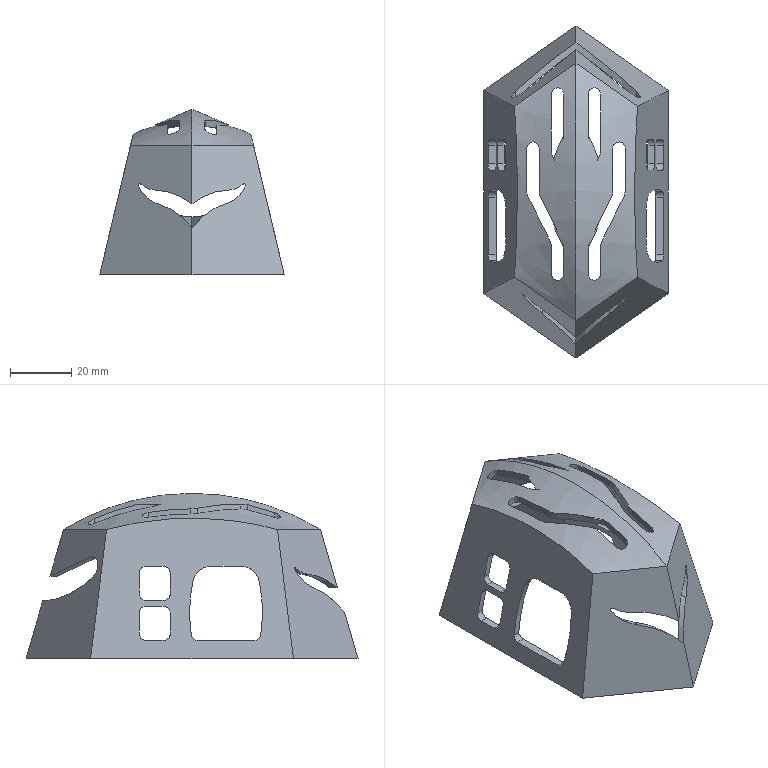Component | NX | SHELL | 1 solid | 134 faces | volume 22662 mm3 | plane 59 | cylinder 57 | spline 18 | commonest cylinder face diameters 4 x26 10 x8 40 x4 12 x4 100 x4 8 x2 0.4 x2 16 x2